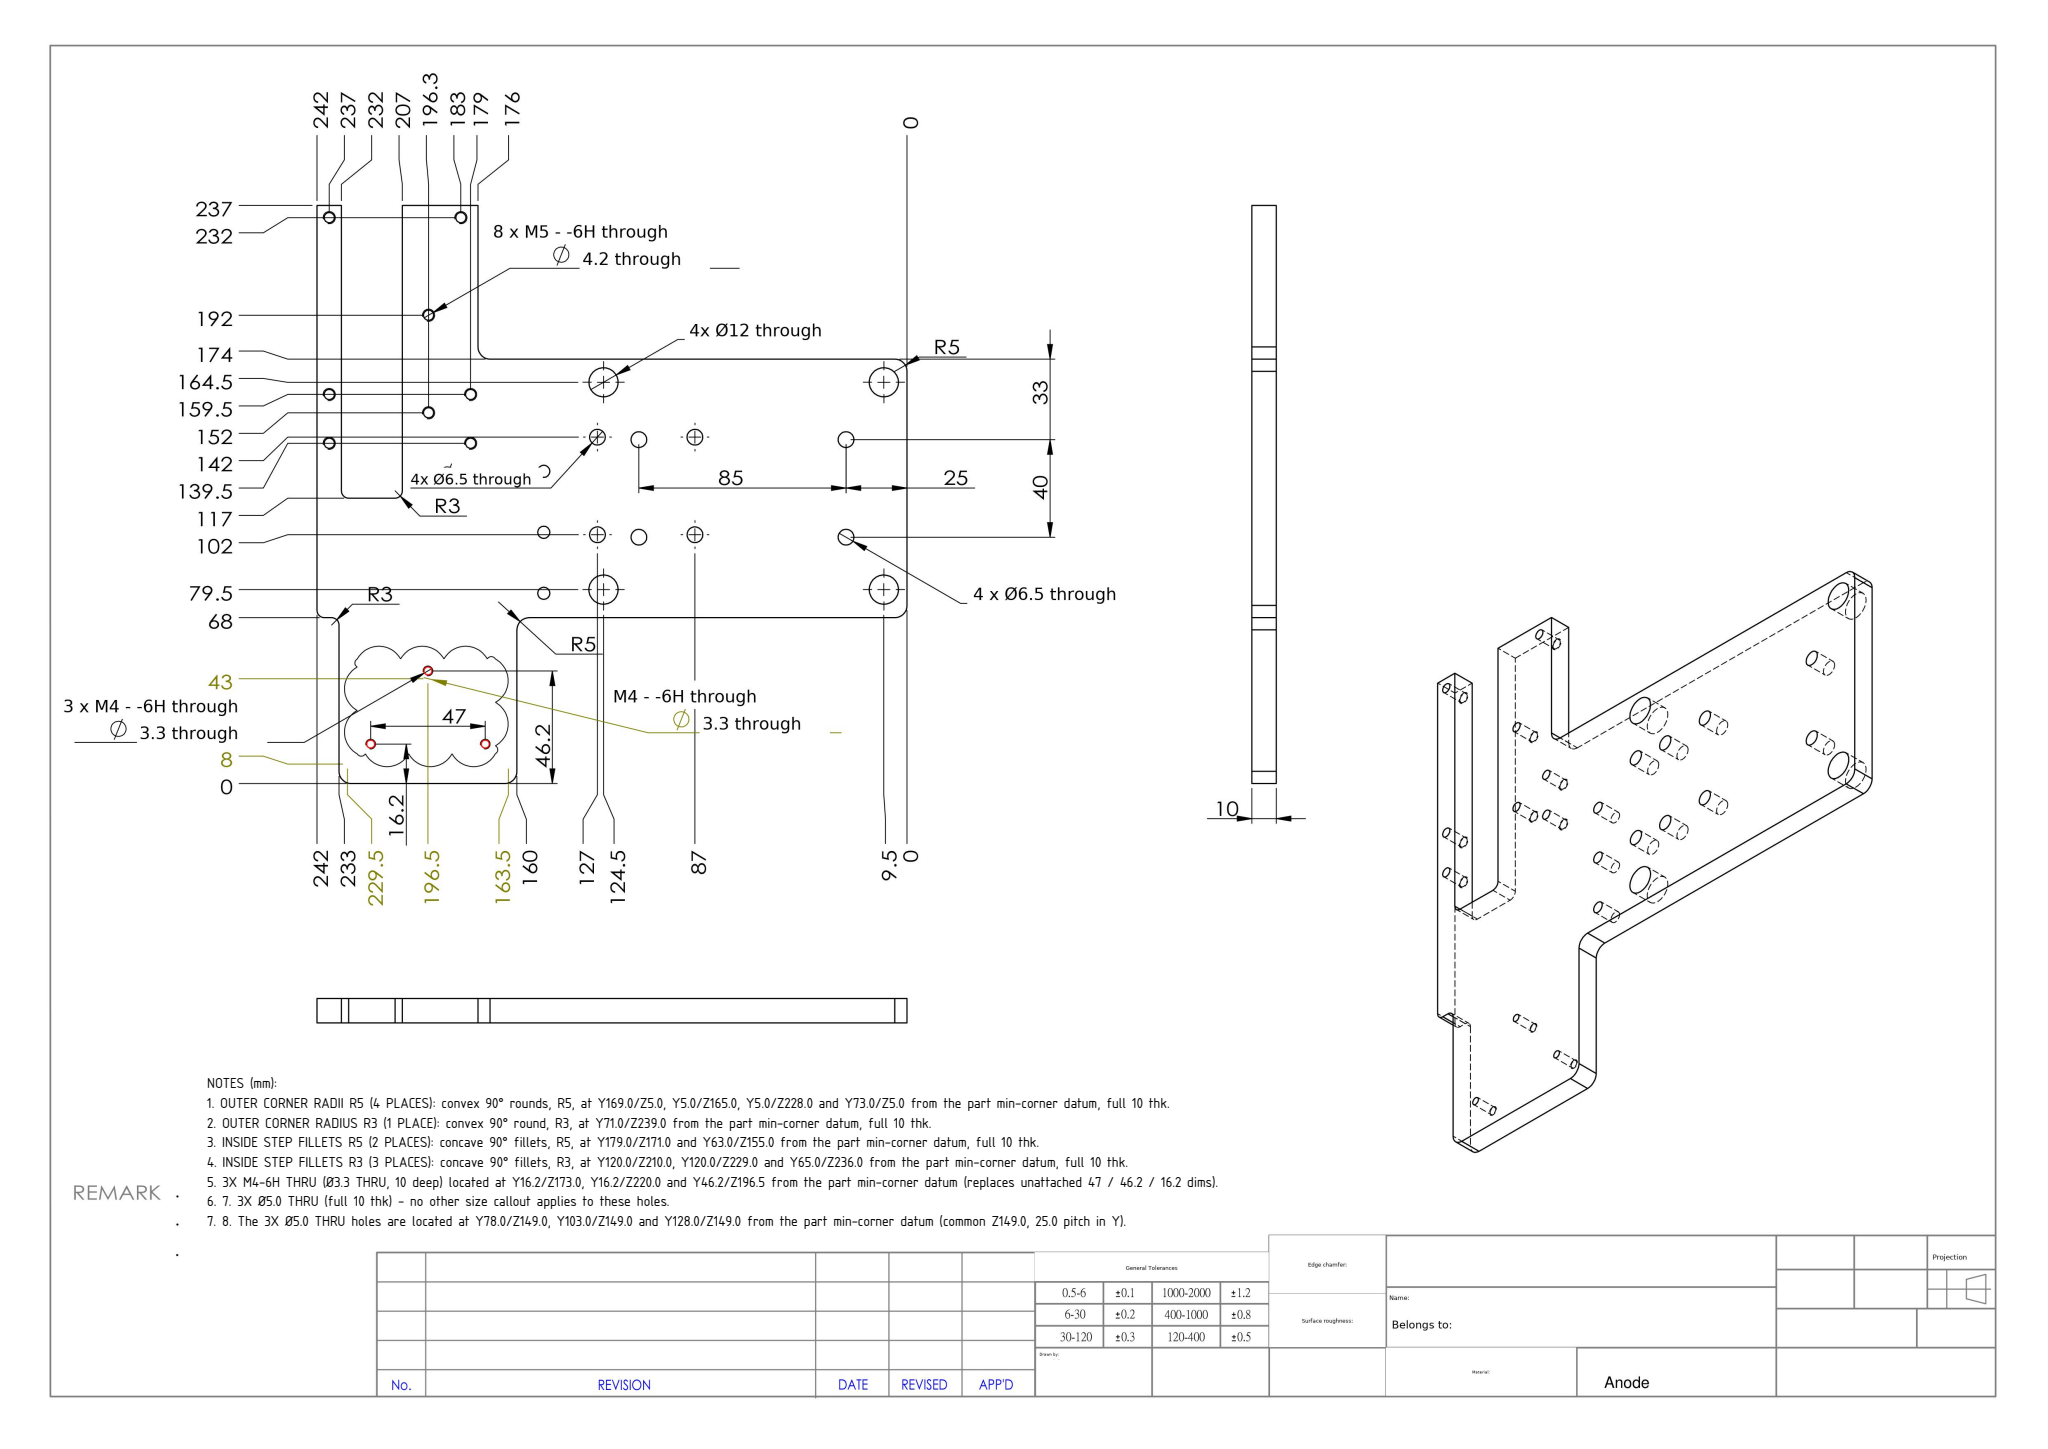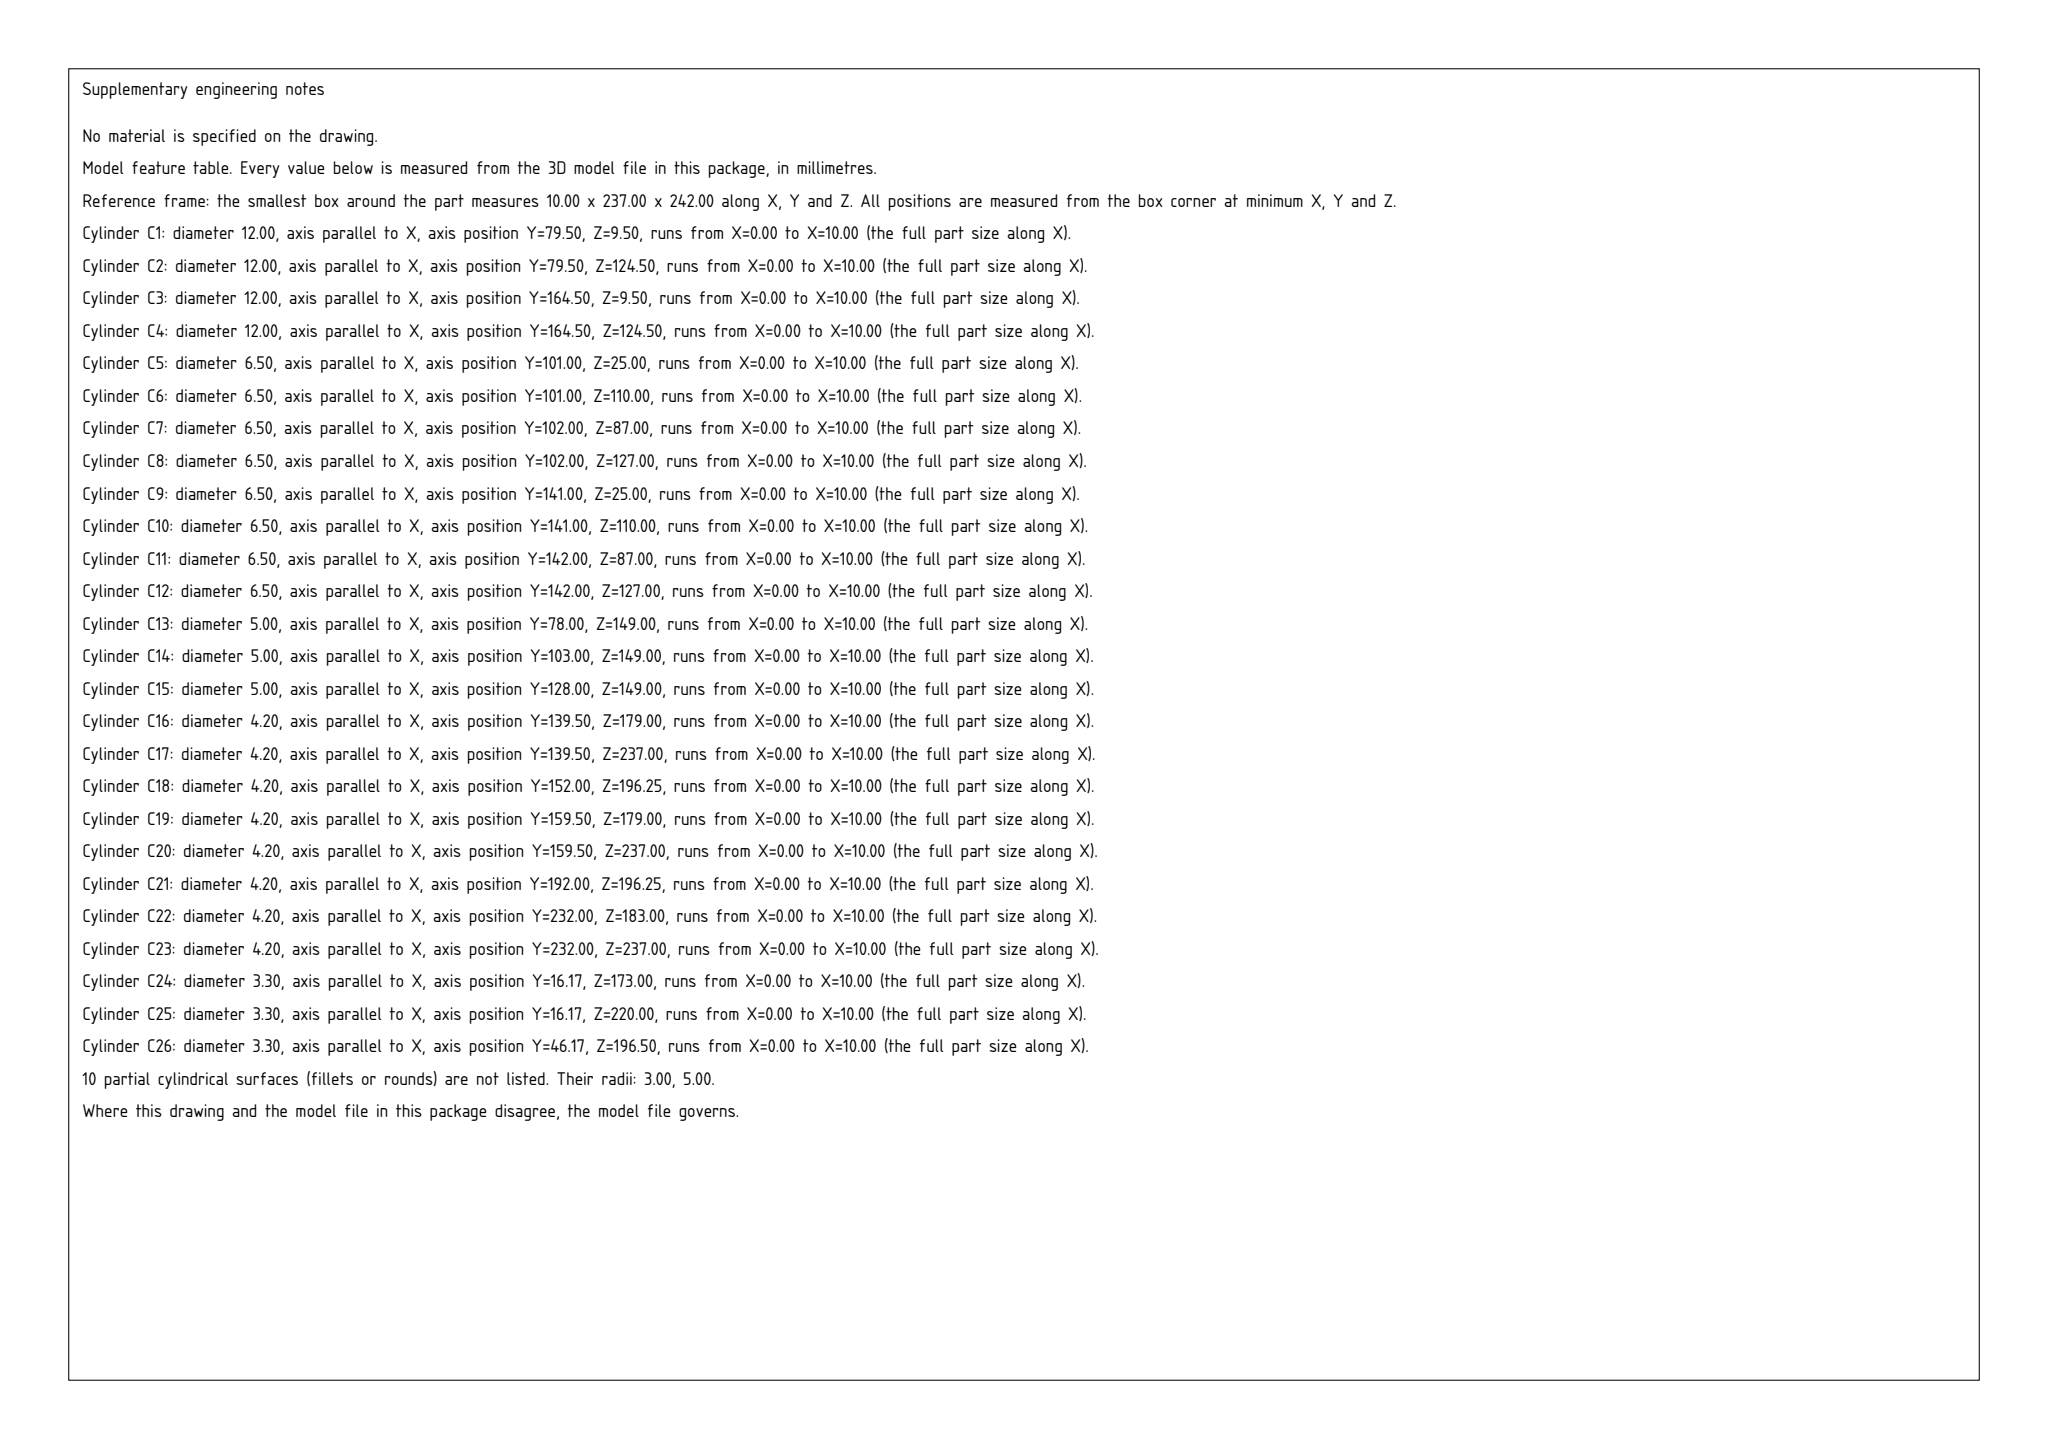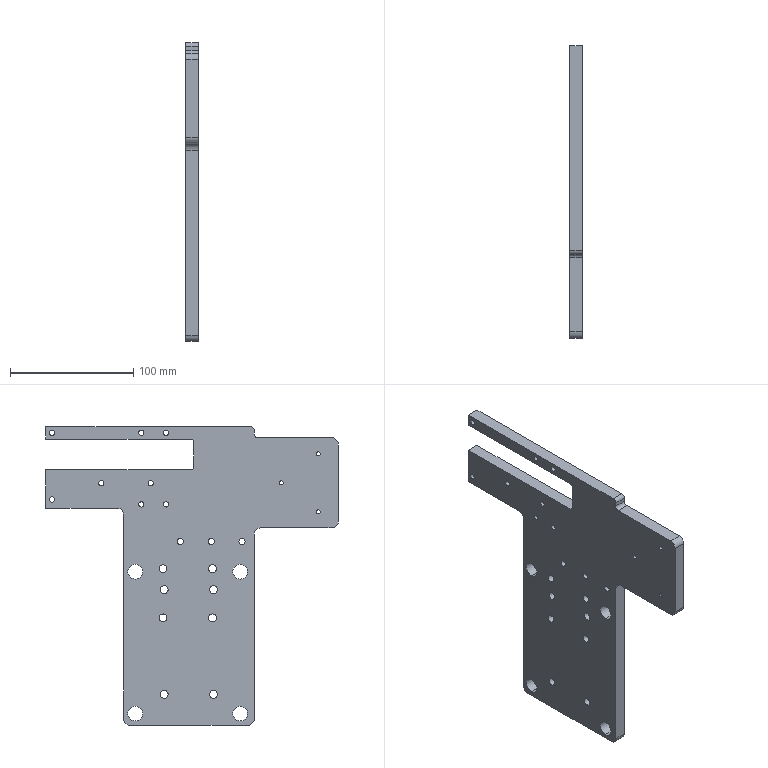Part | SolidWorks | mm | 1 solid | 78 faces | box 10 x 237 x 242 mm | volume 308539 mm3 | cylinder 62 | plane 16 | commonest cylinder face diameters 6.5 x16 4.2 x16 12 x8 5 x6 3.3 x6 10 x6 6 x4
Drawing notes:
OUTER CORNER RADII R5 (4 PLACES): convex 90° rounds, R5, at Y169.0/Z5.0, Y5.0/Z165.0, Y5.0/Z228.0 and Y73.0/Z5.0 from the part min-corner datum, full 10 thk. | from the solid: cylinders: convex arc (round/outer radius) dia 10.0, axis x, at (y,z) = (169,5), (5,165), (5,228), (73,5), from 0.0 to 10.0, arc 90°
OUTER CORNER RADIUS R3 (1 PLACE): convex 90° round, R3, at Y71.0/Z239.0 from the part min-corner datum, full 10 thk. | from the solid: cylinders: convex arc (round/outer radius) dia 6.0, axis x, at (y,z) = (71,239), from 0.0 to 10.0, arc 90°
INSIDE STEP FILLETS R5 (2 PLACES): concave 90° fillets, R5, at Y179.0/Z171.0 and Y63.0/Z155.0 from the part min-corner datum, full 10 thk. | from the solid: cylinders: concave arc (fillet) dia 10.0, axis x, at (y,z) = (179,171) and (63,155), from 0.0 to 10.0, arc 90°
INSIDE STEP FILLETS R3 (3 PLACES): concave 90° fillets, R3, at Y120.0/Z210.0, Y120.0/Z229.0 and Y65.0/Z236.0 from the part min-corner datum, full 10 thk. | from the solid: cylinders: concave arc (fillet) dia 6.0, axis x, at (y,z) = (120,210), (120,229), (65,236), from 0.0 to 10.0, arc 90°
3X M4-6H THRU (Ø3.3 THRU, 10 deep) located at Y16.2/Z173.0, Y16.2/Z220.0 and Y46.2/Z196.5 from the part min-corner datum (replaces unattached 47 / 46.2 / 16.2 dims). | from the solid: cylinders: hole/bore dia 3.3, axis x, at (y,z) = (16.2,173.0), (16.2,220.0), (46.2,196.5), from 0.0 to 10.0, arc 360°
7. 3X Ø5.0 THRU (full 10 thk) - no other size callout applies to these holes. | from the solid: cylinders: hole/bore dia 5.0, axis x, from 0.0 to 10.0, 360 deg (3 instances)
8. The 3X Ø5.0 THRU holes are located at Y78.0/Z149.0, Y103.0/Z149.0 and Y128.0/Z149.0 from the part min-corner datum (common Z149.0, 25.0 pitch in Y). | from the solid: cylinders: hole/bore dia 5.0 at axis_pos (y103.0,z149.0), (y128.0,z149.0), (y78.0,z149.0)
build123d program:
from build123d import *
from OCP.BRepFilletAPI import BRepFilletAPI_MakeFillet

# Parameters (mm, degrees)
SKETCH1_W                  = 290
SKETCH1_H                  = 210
BOSS_EXTRUDE1_DEPTH        = 10
SKETCH2_R                  = 6
CUT_EXTRUDE1_DEPTH         = 180.304
SKETCH7_R                  = 3.25
CUT_EXTRUDE3_DEPTH         = 10
SKETCH8_W                  = 25
SKETCH8_H                  = 100
CUT_EXTRUDE4_DEPTH         = 180.304
SKETCH14_W                 = 10
SKETCH14_H                 = 290
BOSS_EXTRUDE2_DEPTH        = 17
CUT_EXTRUDE5_DEPTH         = 10
CUT_EXTRUDE6_DEPTH         = 10
SKETCH29_W                 = 25
SKETCH29_H                 = 10
CUT_EXTRUDE7_DEPTH         = 10
FILLET1_R1                 = 5
FILLET1_R2                 = 3
SKETCH30_W                 = 10
SKETCH30_H                 = 31
SKETCH30_H_2               = 10
BOSS_EXTRUDE3_DEPTH        = 10
M5_TAPPED_HOLE5_D          = 4.2
M4_TAPPED_HOLE2_D          = 3.3
SKETCH33_R                 = 2.5
CUT_EXTRUDE8_DEPTH         = 186.968
F_6_5_6_5_DIAMETER_HOLE1_D = 6.5


with BuildPart() as part:
    # Sketch1 → Boss-Extrude1 (new body)
    with BuildSketch(Plane(origin=(0, 0, 0), x_dir=(0, 0, -1), z_dir=(1, 0, 0))):
        Rectangle(SKETCH1_W, SKETCH1_H)
    extrude(amount=BOSS_EXTRUDE1_DEPTH)

    # Sketch2 → Cut-Extrude1 (cut, through all)
    with BuildSketch(Plane(origin=(10, 0, 0), x_dir=(0, 0, -1), z_dir=(1, 0, 0))):
        with Locations((92.5, 42.5)):
            Circle(SKETCH2_R)
        with Locations(Location((-22.5, 42.5, 0), (0, 0, 180))):
            Circle(SKETCH2_R)
        with Locations((-22.5, -42.5)):
            Circle(SKETCH2_R)
        with Locations(Location((92.5, -42.5, 0), (0, 0, 180))):
            Circle(SKETCH2_R)
    extrude(amount=-CUT_EXTRUDE1_DEPTH, mode=Mode.SUBTRACT)

    # Sketch7 → Cut-Extrude3 (cut)
    with BuildSketch(Plane(origin=(10, 0, 0), x_dir=(0, 0, -1), z_dir=(1, 0, 0))):
        with Locations((-25, 20)):
            Circle(SKETCH7_R)
        with Locations(Location((15, 20, 0), (0, 0, 180))):
            Circle(SKETCH7_R)
        with Locations((15, -20)):
            Circle(SKETCH7_R)
        with Locations(Location((-25, -20, 0), (0, 0, 180))):
            Circle(SKETCH7_R)
    extrude(amount=-CUT_EXTRUDE3_DEPTH, mode=Mode.SUBTRACT)

    # Sketch8 → Cut-Extrude4 (cut, through all)
    with BuildSketch(Plane(origin=(10, 0, 0), x_dir=(0, 0, -1), z_dir=(1, 0, 0))):
        with Locations((-117.5, 55)):
            Rectangle(SKETCH8_W, SKETCH8_H)
    extrude(amount=-CUT_EXTRUDE4_DEPTH, mode=Mode.SUBTRACT)

    # Sketch14 → Boss-Extrude2 (add)
    with BuildSketch(Plane.XZ.offset(105)):
        with Locations((5, 0)):
            Rectangle(SKETCH14_W, SKETCH14_H)
    extrude(amount=BOSS_EXTRUDE2_DEPTH)

    # Sketch19 → Cut-Extrude5 (cut)
    with BuildSketch(Plane.ZY):
        Polygon((-145, 105), (55, 105), (55, 60), (-110, 60), (-110, -72), (45, -72), (45, -122), (-145, -122), (-145, -72), (-145, 60), align=None)
    extrude(amount=-CUT_EXTRUDE5_DEPTH, mode=Mode.SUBTRACT)

    # Sketch26 → Cut-Extrude6 (cut)
    with BuildSketch(Plane.ZY):
        Polygon((-110, 60), (-110, -72), (-100, -72), (45, -72), (45, -122), (58, -122), (58, -54), (45, -54), (-102, -54), (-102, 52), (55, 52), (74, 52), (74, 105), (55, 105), (55, 60), align=None)
        Polygon((140, -122), (131, -122), (131, -54), (140, -54), (140, 105), (145, 105), (145, -122), align=None)
    extrude(amount=-CUT_EXTRUDE6_DEPTH, mode=Mode.SUBTRACT)

    # Sketch29 → Cut-Extrude7 (cut)
    with BuildSketch(Plane.ZY):
        with Locations((117.5, 0)):
            Rectangle(SKETCH29_W, SKETCH29_H)
    extrude(amount=-CUT_EXTRUDE7_DEPTH, mode=Mode.SUBTRACT)

    # Fillet1: one fillet with a radius per group of edges: ONE call of the kernel's fillet builder (fillet() takes one radius for all edges)
    fillet1_edges_1 = [part.edges().sort_by_distance(p)[0] for p in [
        (5, -54, -102),
        (5, 52, -102),
        (5, 52, 74),
        (5, -122, 131),
        (5, -54, 58),
        (5, -122, 58),
    ]]
    fillet1_edges_2 = [part.edges().sort_by_distance(p)[0] for p in [
        (5, -54, 131),
        (5, -54, 140),
        (5, -5, 130),
        (5, -5, 105),
    ]]
    fillet1 = BRepFilletAPI_MakeFillet(part.part.solid().wrapped)
    for e in fillet1_edges_1:
        fillet1.Add(FILLET1_R1, e.wrapped)
    for e in fillet1_edges_2:
        fillet1.Add(FILLET1_R2, e.wrapped)
    add(Compound.cast(fillet1.Shape()), mode=Mode.REPLACE)

    # Sketch30 → Boss-Extrude3 (add)
    with BuildSketch(Plane(origin=(0, 105, 0), x_dir=(1, 0, 0), z_dir=(0, 1, 0))):
        with Locations((5, -89.5)):
            Rectangle(SKETCH30_W, SKETCH30_H)
        with Locations((5, -135)):
            Rectangle(SKETCH30_W, SKETCH30_H_2)
    extrude(amount=BOSS_EXTRUDE3_DEPTH)

    # M5 Tapped Hole5 (through all)
    with Locations(Plane.ZY):
        with Locations((94.25, 30), (135, 17.5), (135, 37.5), (77, 37.5), (77, 17.5), (94.25, 70), (81, 110), (135, 110)):
            Hole(M5_TAPPED_HOLE5_D / 2)

    # M4 Tapped Hole2 (through all)
    with Locations(Plane.ZY):
        with Locations((71, -105.832), (94.5, -75.832), (118, -105.832)):
            Hole(M4_TAPPED_HOLE2_D / 2)

    # Sketch33 → Cut-Extrude8 (cut, through all)
    with BuildSketch(Plane(origin=(10, 0, 0), x_dir=(0, 0, -1), z_dir=(1, 0, 0))):
        with Locations((-47, -44)):
            Circle(SKETCH33_R)
        with Locations((-47, -19)):
            Circle(SKETCH33_R)
        with Locations((-47, 6)):
            Circle(SKETCH33_R)
    extrude(amount=-CUT_EXTRUDE8_DEPTH, mode=Mode.SUBTRACT)

    # 6.5 _6.5_ Diameter Hole1 (through all)
    with Locations(Plane(origin=(10, 0, 0), x_dir=(0, 0, -1), z_dir=(1, 0, 0))):
        with Locations((77, 19), (77, -21), (-8, -21), (-8, 19)):
            Hole(F_6_5_6_5_DIAMETER_HOLE1_D / 2)


solid = part.part